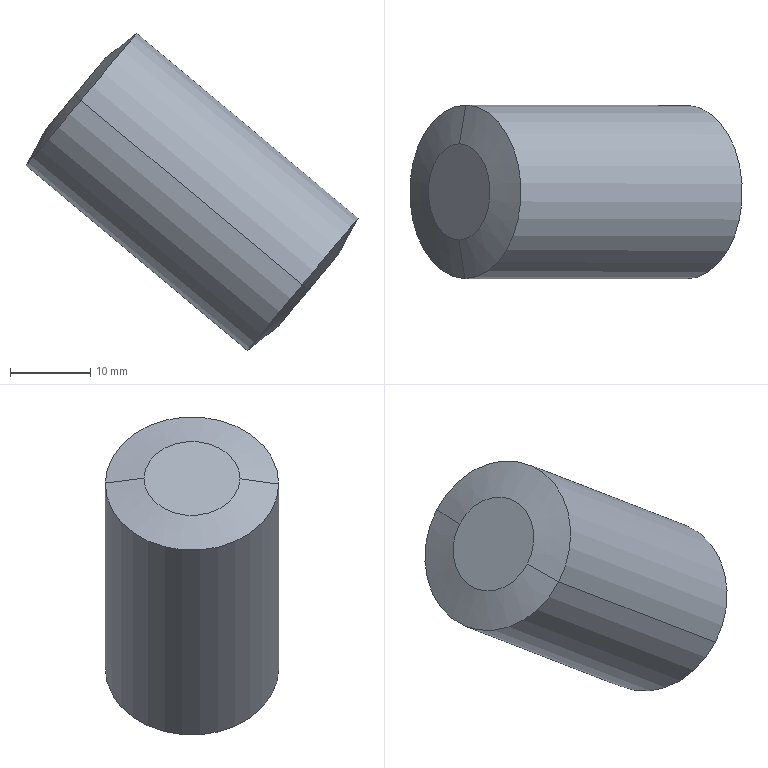Component | SolidWorks | 30-01A-1_Wheel-322-1_CJH65-322-1_CJH65bearing-322-1 | 1 solid | 8 faces | box 41.52 x 21.67 x 39.71 mm | volume 13731 mm3 | cone 4 | cylinder 2 | plane 2 | commonest cylinder face diameters 21.667 x2
build123d program:
from build123d import *


with BuildPart() as part:
    # Sketch1 → Revolve1 (revolve)
    with BuildSketch(Plane.XY, mode=Mode.PRIVATE) as revolve1_sk:
        Polygon((-19, 0), (-19, 6), (-18, 10.833), (18, 10.833), (19, 6), (19, 0), align=None)
    revolve(revolve1_sk.sketch.rotate(Axis((19, 0, 0), (-1, 0, 0)), 270), axis=Axis((19, 0, 0), (-1, 0, 0)))


solid = part.part

# Placed as in the assembly
solid = solid.moved(Location((177.3, -622.345, -91.473), (-98.879, -7.345, 39.294)))
STEP:
#1=CARTESIAN_POINT('',(6.407,-24.266,-3.12));
#2=VERTEX_POINT('',#1);
#3=CARTESIAN_POINT('',(6.405,-24.738,-3.123));
#4=VERTEX_POINT('',#3);
#5=CARTESIAN_POINT('',(6.406,-24.502,-3.122));
#6=DIRECTION('',(0.7676,-0.,-0.641));
#7=DIRECTION('',(0.00514,1.,0.006155));
#8=AXIS2_PLACEMENT_3D('',#5,#6,#7);
#9=CIRCLE('',#8,0.2362);
#10=EDGE_CURVE('',#2,#4,#9,.T.);
#11=ORIENTED_EDGE('',*,*,#10,.T.);
#12=CARTESIAN_POINT('',(6.434,-24.928,-3.15));
#13=VERTEX_POINT('',#12);
#14=CARTESIAN_POINT('',(6.405,-24.738,-3.123));
#15=DIRECTION('',(0.1505,-0.9792,-0.1359));
#16=VECTOR('',#15,39.37);
#17=LINE('',#14,#16);
#18=EDGE_CURVE('',#4,#13,#17,.T.);
#19=ORIENTED_EDGE('',*,*,#18,.T.);
#20=CARTESIAN_POINT('',(6.439,-24.075,-3.144));
#21=VERTEX_POINT('',#20);
#22=CARTESIAN_POINT('',(6.436,-24.502,-3.147));
#23=DIRECTION('',(0.7676,-0.,-0.641));
#24=DIRECTION('',(0.00514,1.,0.006155));
#25=AXIS2_PLACEMENT_3D('',#22,#23,#24);
#26=CIRCLE('',#25,0.4265);
#27=EDGE_CURVE('',#21,#13,#26,.T.);
#28=ORIENTED_EDGE('',*,*,#27,.F.);
#29=CARTESIAN_POINT('',(6.407,-24.266,-3.12));
#30=DIRECTION('',(0.1605,0.9792,-0.1238));
#31=VECTOR('',#30,39.37);
#32=LINE('',#29,#31);
#33=EDGE_CURVE('',#2,#21,#32,.T.);
#34=ORIENTED_EDGE('',*,*,#33,.F.);
#35=EDGE_LOOP('',(#11,#19,#28,#34));
#36=FACE_OUTER_BOUND('',#35,.T.);
#37=CARTESIAN_POINT('',(6.406,-24.502,-3.122));
#38=DIRECTION('',(0.7676,-0.,-0.641));
#39=DIRECTION('',(0.00514,1.,0.006155));
#40=AXIS2_PLACEMENT_3D('',#37,#38,#39);
#41=CONICAL_SURFACE('',#40,0.2362,1.367);
#42=ADVANCED_FACE('',(#36),#41,.T.);
#43=ORIENTED_EDGE('',*,*,#27,.T.);
#44=CARTESIAN_POINT('',(7.522,-24.928,-4.058));
#45=VERTEX_POINT('',#44);
#46=CARTESIAN_POINT('',(6.404,-24.928,-3.124));
#47=DIRECTION('',(0.7676,-0.,-0.641));
#48=VECTOR('',#47,39.37);
#49=LINE('',#46,#48);
#50=EDGE_CURVE('',#13,#45,#49,.T.);
#51=ORIENTED_EDGE('',*,*,#50,.T.);
#52=CARTESIAN_POINT('',(7.526,-24.075,-4.053));
#53=VERTEX_POINT('',#52);
#54=CARTESIAN_POINT('',(7.524,-24.502,-4.056));
#55=DIRECTION('',(0.7676,-0.,-0.641));
#56=DIRECTION('',(0.00514,1.,0.006155));
#57=AXIS2_PLACEMENT_3D('',#54,#55,#56);
#58=CIRCLE('',#57,0.4265);
#59=EDGE_CURVE('',#53,#45,#58,.T.);
#60=ORIENTED_EDGE('',*,*,#59,.F.);
#61=CARTESIAN_POINT('',(6.408,-24.075,-3.119));
#62=DIRECTION('',(0.7676,-0.,-0.641));
#63=VECTOR('',#62,39.37);
#64=LINE('',#61,#63);
#65=EDGE_CURVE('',#21,#53,#64,.T.);
#66=ORIENTED_EDGE('',*,*,#65,.F.);
#67=EDGE_LOOP('',(#43,#51,#60,#66));
#68=FACE_OUTER_BOUND('',#67,.T.);
#69=CARTESIAN_POINT('',(6.406,-24.502,-3.122));
#70=DIRECTION('',(0.7676,-0.,-0.641));
#71=DIRECTION('',(0.00514,1.,0.006155));
#72=AXIS2_PLACEMENT_3D('',#69,#70,#71);
#73=CYLINDRICAL_SURFACE('',#72,0.4265);
#74=ADVANCED_FACE('',(#68),#73,.T.);
#75=CARTESIAN_POINT('',(7.556,-24.266,-4.079));
#76=VERTEX_POINT('',#75);
#77=CARTESIAN_POINT('',(7.553,-24.738,-4.082));
#78=VERTEX_POINT('',#77);
#79=CARTESIAN_POINT('',(7.554,-24.502,-4.081));
#80=DIRECTION('',(0.7676,-0.,-0.641));
#81=DIRECTION('',(0.00514,1.,0.006155));
#82=AXIS2_PLACEMENT_3D('',#79,#80,#81);
#83=CIRCLE('',#82,0.2362);
#84=EDGE_CURVE('',#76,#78,#83,.T.);
#85=ORIENTED_EDGE('',*,*,#84,.F.);
#86=CARTESIAN_POINT('',(7.526,-24.075,-4.053));
#87=DIRECTION('',(-0.1505,0.9792,0.1359));
#88=VECTOR('',#87,39.37);
#89=LINE('',#86,#88);
#90=EDGE_CURVE('',#76,#53,#89,.T.);
#91=ORIENTED_EDGE('',*,*,#90,.T.);
#92=ORIENTED_EDGE('',*,*,#59,.T.);
#93=CARTESIAN_POINT('',(7.522,-24.928,-4.058));
#94=DIRECTION('',(-0.1605,-0.9792,0.1238));
#95=VECTOR('',#94,39.37);
#96=LINE('',#93,#95);
#97=EDGE_CURVE('',#78,#45,#96,.T.);
#98=ORIENTED_EDGE('',*,*,#97,.F.);
#99=EDGE_LOOP('',(#85,#91,#92,#98));
#100=FACE_OUTER_BOUND('',#99,.T.);
#101=CARTESIAN_POINT('',(7.524,-24.502,-4.056));
#102=DIRECTION('',(-0.7676,0.,0.641));
#103=DIRECTION('',(-0.00514,-1.,-0.006155));
#104=AXIS2_PLACEMENT_3D('',#101,#102,#103);
#105=CONICAL_SURFACE('',#104,0.4265,1.367);
#106=ADVANCED_FACE('',(#100),#105,.T.);
#107=CARTESIAN_POINT('',(7.554,-24.502,-4.081));
#108=DIRECTION('',(0.7676,-0.,-0.641));
#109=DIRECTION('',(0.00514,1.,0.006155));
#110=AXIS2_PLACEMENT_3D('',#107,#108,#109);
#111=CIRCLE('',#110,0.2362);
#112=EDGE_CURVE('',#78,#76,#111,.T.);
#113=ORIENTED_EDGE('',*,*,#112,.T.);
#114=ORIENTED_EDGE('',*,*,#84,.T.);
#115=EDGE_LOOP('',(#113,#114));
#116=FACE_OUTER_BOUND('',#115,.T.);
#117=CARTESIAN_POINT('',(7.554,-24.502,-4.081));
#118=DIRECTION('',(-0.7676,0.,0.641));
#119=DIRECTION('',(-0.00514,-1.,-0.006155));
#120=AXIS2_PLACEMENT_3D('',#117,#118,#119);
#121=PLANE('',#120);
#122=ADVANCED_FACE('',(#116),#121,.F.);
#123=ORIENTED_EDGE('',*,*,#90,.F.);
#124=ORIENTED_EDGE('',*,*,#112,.F.);
#125=ORIENTED_EDGE('',*,*,#97,.T.);
#126=CARTESIAN_POINT('',(7.524,-24.502,-4.056));
#127=DIRECTION('',(0.7676,-0.,-0.641));
#128=DIRECTION('',(0.00514,1.,0.006155));
#129=AXIS2_PLACEMENT_3D('',#126,#127,#128);
#130=CIRCLE('',#129,0.4265);
#131=EDGE_CURVE('',#45,#53,#130,.T.);
#132=ORIENTED_EDGE('',*,*,#131,.T.);
#133=EDGE_LOOP('',(#123,#124,#125,#132));
#134=FACE_OUTER_BOUND('',#133,.T.);
#135=CARTESIAN_POINT('',(7.524,-24.502,-4.056));
#136=DIRECTION('',(-0.7676,0.,0.641));
#137=DIRECTION('',(-0.00514,-1.,-0.006155));
#138=AXIS2_PLACEMENT_3D('',#135,#136,#137);
#139=CONICAL_SURFACE('',#138,0.4265,1.367);
#140=ADVANCED_FACE('',(#134),#139,.T.);
#141=ORIENTED_EDGE('',*,*,#50,.F.);
#142=CARTESIAN_POINT('',(6.436,-24.502,-3.147));
#143=DIRECTION('',(0.7676,-0.,-0.641));
#144=DIRECTION('',(0.00514,1.,0.006155));
#145=AXIS2_PLACEMENT_3D('',#142,#143,#144);
#146=CIRCLE('',#145,0.4265);
#147=EDGE_CURVE('',#13,#21,#146,.T.);
#148=ORIENTED_EDGE('',*,*,#147,.T.);
#149=ORIENTED_EDGE('',*,*,#65,.T.);
#150=ORIENTED_EDGE('',*,*,#131,.F.);
#151=EDGE_LOOP('',(#141,#148,#149,#150));
#152=FACE_OUTER_BOUND('',#151,.T.);
#153=CARTESIAN_POINT('',(6.406,-24.502,-3.122));
#154=DIRECTION('',(0.7676,-0.,-0.641));
#155=DIRECTION('',(0.00514,1.,0.006155));
#156=AXIS2_PLACEMENT_3D('',#153,#154,#155);
#157=CYLINDRICAL_SURFACE('',#156,0.4265);
#158=ADVANCED_FACE('',(#152),#157,.T.);
#159=ORIENTED_EDGE('',*,*,#18,.F.);
#160=CARTESIAN_POINT('',(6.406,-24.502,-3.122));
#161=DIRECTION('',(0.7676,-0.,-0.641));
#162=DIRECTION('',(0.00514,1.,0.006155));
#163=AXIS2_PLACEMENT_3D('',#160,#161,#162);
#164=CIRCLE('',#163,0.2362);
#165=EDGE_CURVE('',#4,#2,#164,.T.);
#166=ORIENTED_EDGE('',*,*,#165,.T.);
#167=ORIENTED_EDGE('',*,*,#33,.T.);
#168=ORIENTED_EDGE('',*,*,#147,.F.);
#169=EDGE_LOOP('',(#159,#166,#167,#168));
#170=FACE_OUTER_BOUND('',#169,.T.);
#171=CARTESIAN_POINT('',(6.406,-24.502,-3.122));
#172=DIRECTION('',(0.7676,-0.,-0.641));
#173=DIRECTION('',(0.00514,1.,0.006155));
#174=AXIS2_PLACEMENT_3D('',#171,#172,#173);
#175=CONICAL_SURFACE('',#174,0.2362,1.367);
#176=ADVANCED_FACE('',(#170),#175,.T.);
#177=ORIENTED_EDGE('',*,*,#10,.F.);
#178=ORIENTED_EDGE('',*,*,#165,.F.);
#179=EDGE_LOOP('',(#177,#178));
#180=FACE_OUTER_BOUND('',#179,.T.);
#181=CARTESIAN_POINT('',(6.558,-24.504,-2.941));
#182=DIRECTION('',(0.7676,-0.,-0.641));
#183=DIRECTION('',(0.00514,1.,0.006155));
#184=AXIS2_PLACEMENT_3D('',#181,#182,#183);
#185=PLANE('',#184);
#186=ADVANCED_FACE('',(#180),#185,.F.);
#187=CLOSED_SHELL('',(#42,#74,#106,#122,#140,#158,#176,#186));
#188=MANIFOLD_SOLID_BREP('',#187);
#189=CARTESIAN_POINT('',(0.,0.,0.));
#190=DIRECTION('',(0.,0.,1.));
#191=DIRECTION('',(1.,0.,0.));
#192=AXIS2_PLACEMENT_3D('',#189,#190,#191);
#193=(LENGTH_UNIT()NAMED_UNIT(*)SI_UNIT($,.METRE.));
#194=LENGTH_MEASURE_WITH_UNIT(LENGTH_MEASURE(0.0254),#193);
#195=DIMENSIONAL_EXPONENTS(1.,0.,0.,0.,0.,0.,0.);
#196=(CONVERSION_BASED_UNIT('',#194)LENGTH_UNIT()NAMED_UNIT(#195));
#197=UNCERTAINTY_MEASURE_WITH_UNIT(LENGTH_MEASURE(0.00001),#196,'','');
#198=(NAMED_UNIT(*)PLANE_ANGLE_UNIT()SI_UNIT($,.RADIAN.));
#199=(NAMED_UNIT(*)SI_UNIT($,.STERADIAN.)SOLID_ANGLE_UNIT());
#200=(GEOMETRIC_REPRESENTATION_CONTEXT(3)GLOBAL_UNCERTAINTY_ASSIGNED_CONTEXT((#197))GLOBAL_UNIT_ASSIGNED_CONTEXT((#196,#198,#199))REPRESENTATION_CONTEXT('',''));
#201=ADVANCED_BREP_SHAPE_REPRESENTATION('',(#188,#192),#200);
#202=COLOUR_RGB('',0.7922,0.8196,0.9333);
#203=FILL_AREA_STYLE_COLOUR('',#202);
#204=FILL_AREA_STYLE('',(#203));
#205=SURFACE_STYLE_FILL_AREA(#204);
#206=SURFACE_SIDE_STYLE('',(#205));
#207=SURFACE_STYLE_USAGE(.BOTH.,#206);
#208=PRESENTATION_STYLE_ASSIGNMENT((#207));
#209=STYLED_ITEM('',(#208),#188);
#210=PRESENTATION_LAYER_ASSIGNMENT('','',(#209));
#211=(LENGTH_UNIT()NAMED_UNIT(*)SI_UNIT($,.METRE.));
#212=LENGTH_MEASURE_WITH_UNIT(LENGTH_MEASURE(0.0254),#211);
#213=DIMENSIONAL_EXPONENTS(1.,0.,0.,0.,0.,0.,0.);
#214=(CONVERSION_BASED_UNIT('',#212)LENGTH_UNIT()NAMED_UNIT(#213));
#215=UNCERTAINTY_MEASURE_WITH_UNIT(LENGTH_MEASURE(0.00001),#214,'','');
#216=(NAMED_UNIT(*)PLANE_ANGLE_UNIT()SI_UNIT($,.RADIAN.));
#217=(NAMED_UNIT(*)SI_UNIT($,.STERADIAN.)SOLID_ANGLE_UNIT());
#218=(GEOMETRIC_REPRESENTATION_CONTEXT(3)GLOBAL_UNCERTAINTY_ASSIGNED_CONTEXT((#215))GLOBAL_UNIT_ASSIGNED_CONTEXT((#214,#216,#217))REPRESENTATION_CONTEXT('',''));
#219=MECHANICAL_DESIGN_GEOMETRIC_PRESENTATION_REPRESENTATION('',(#209),#218);